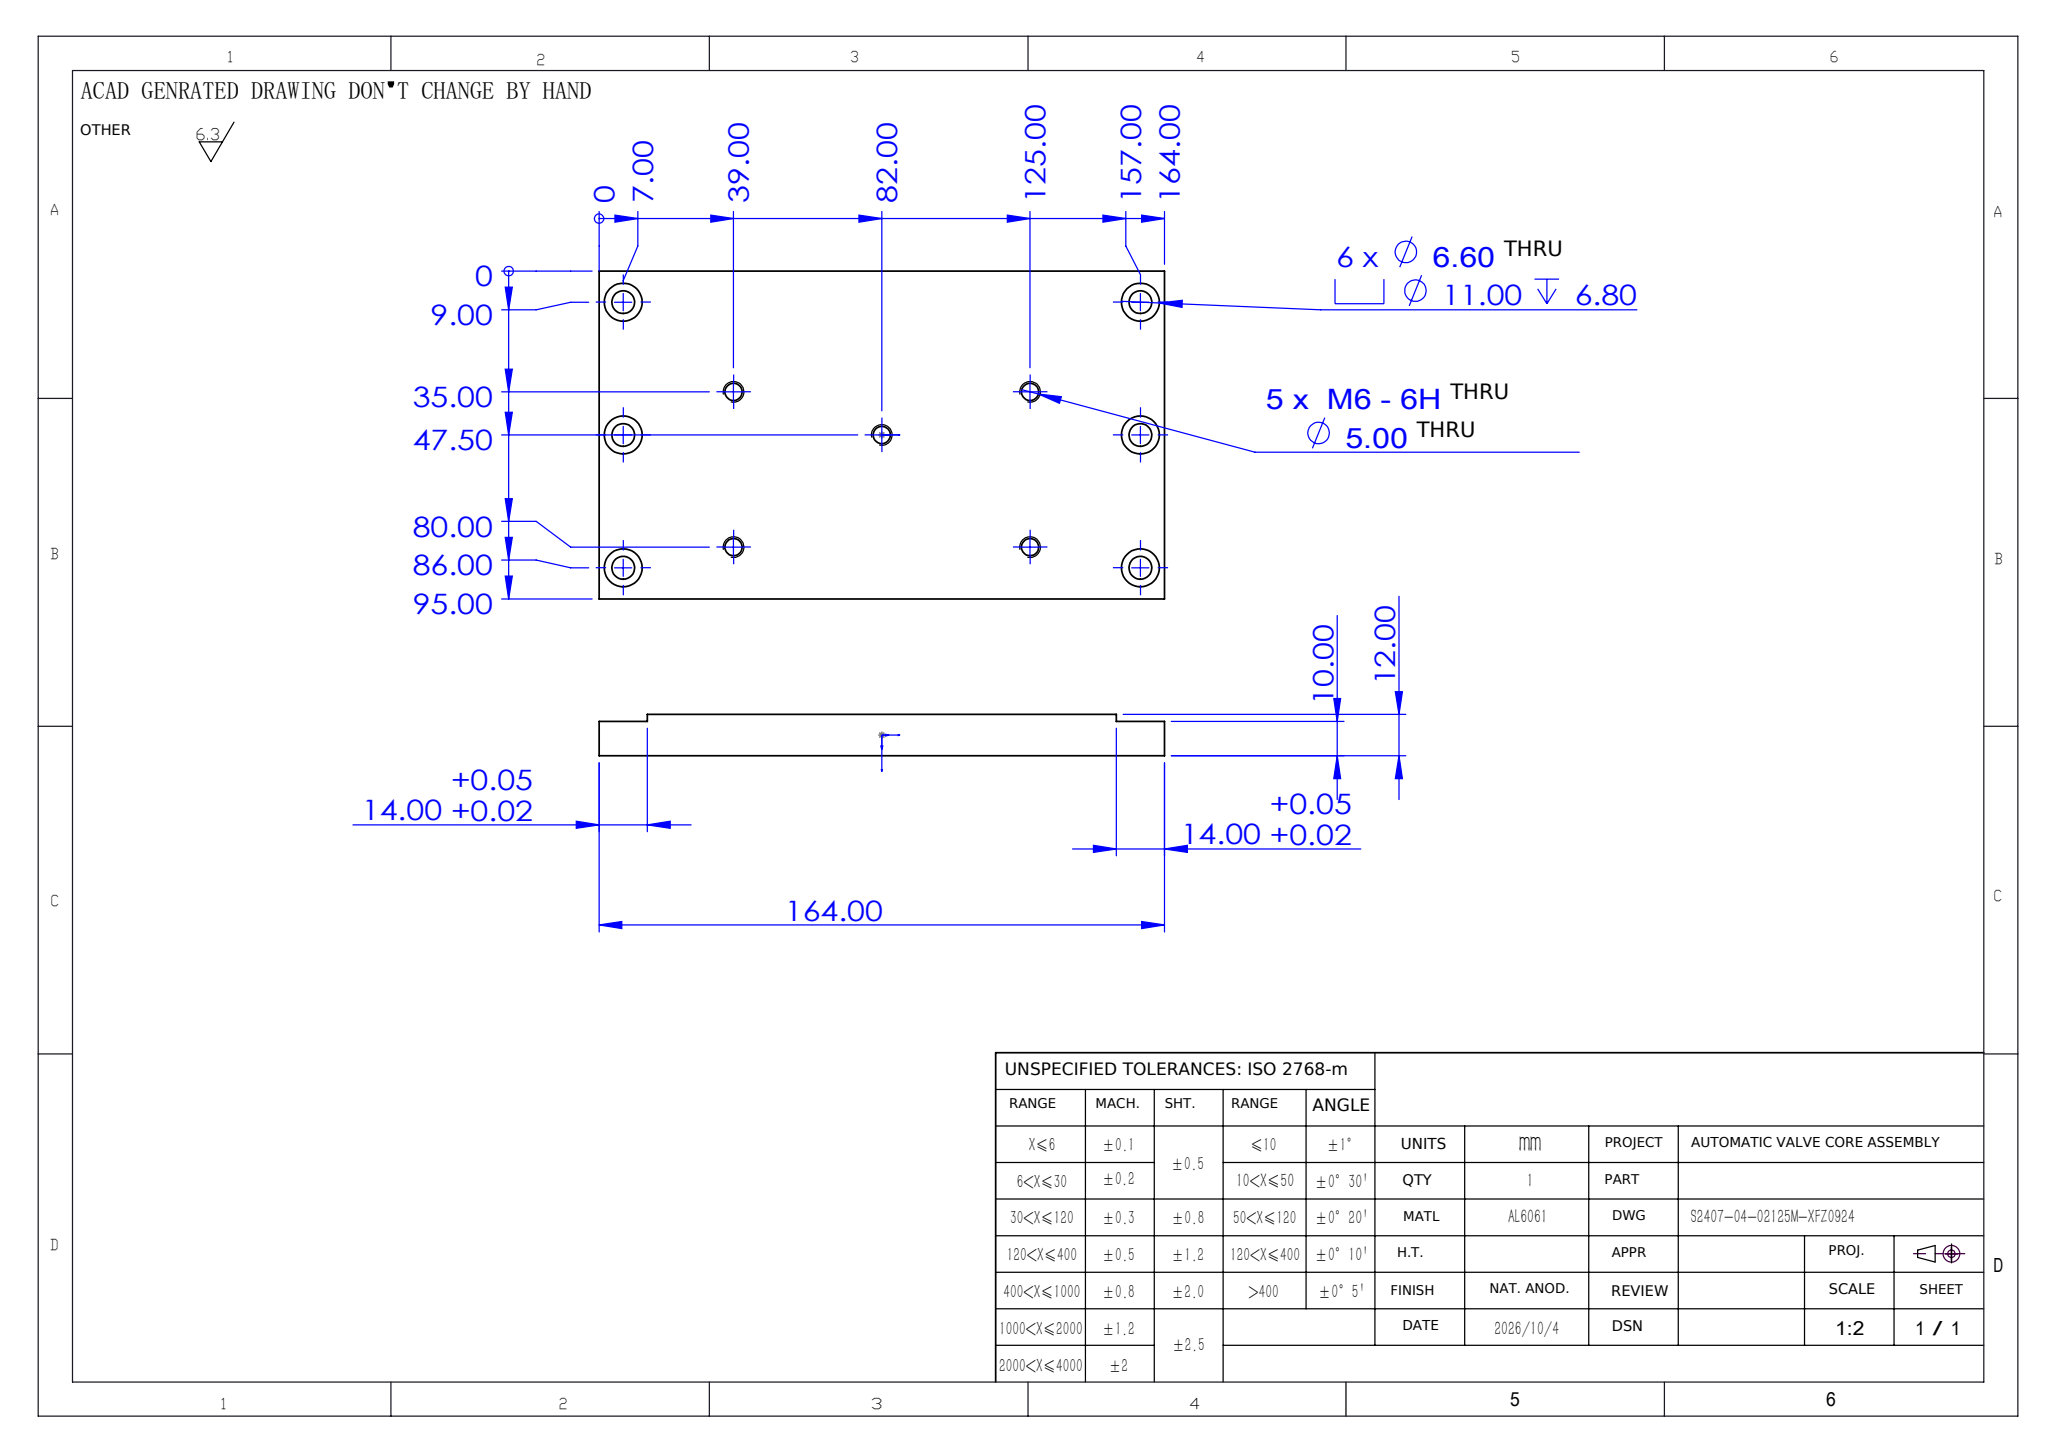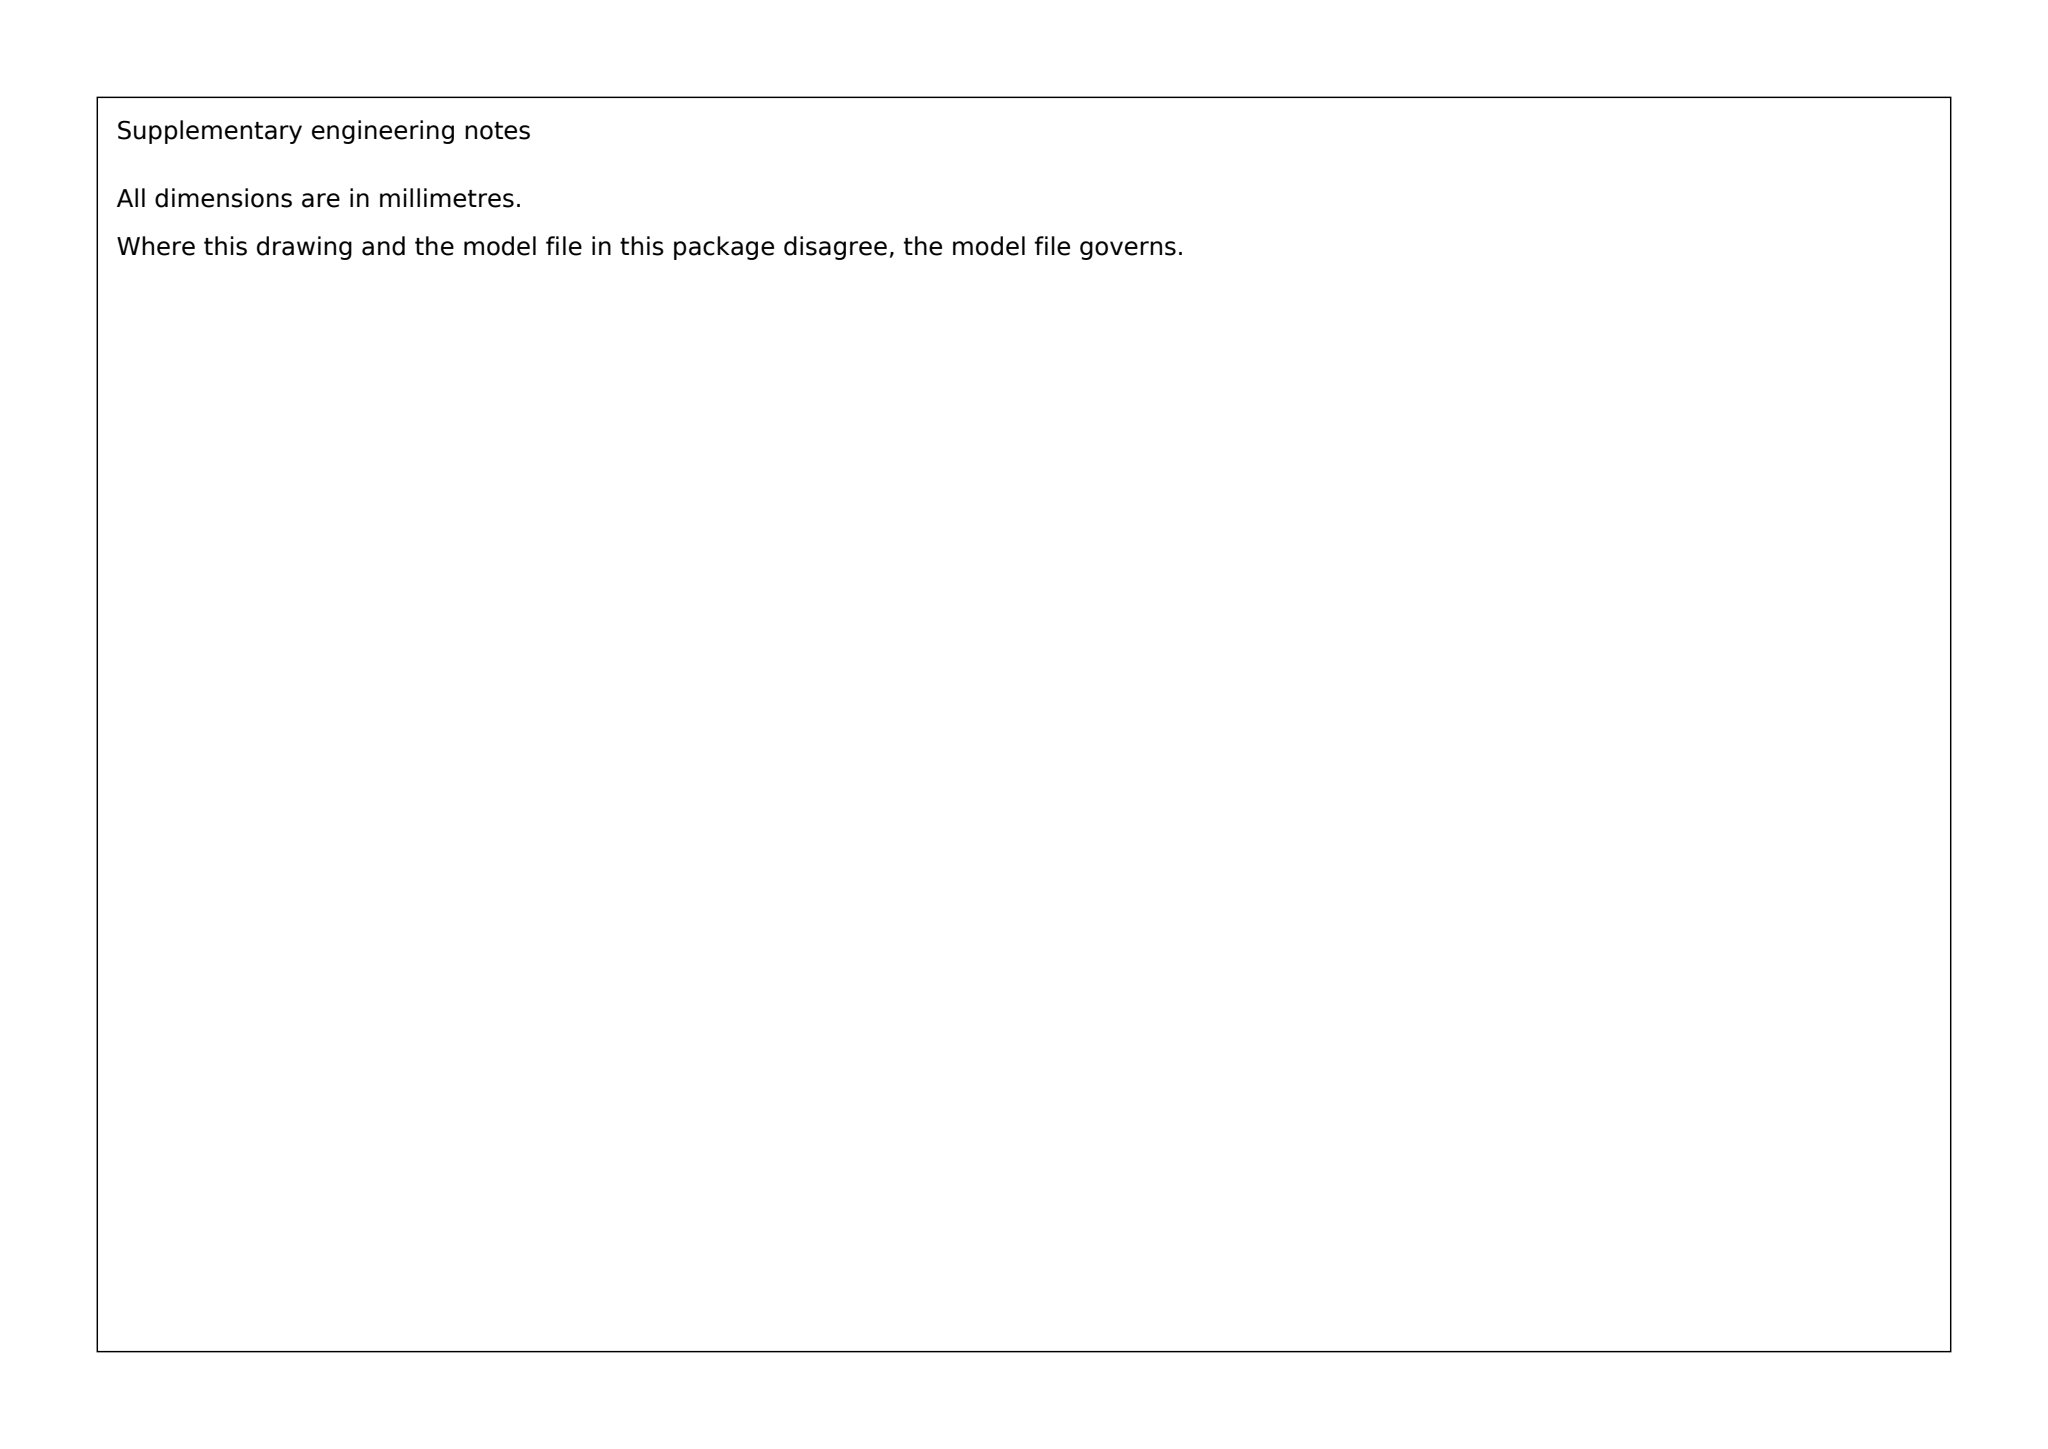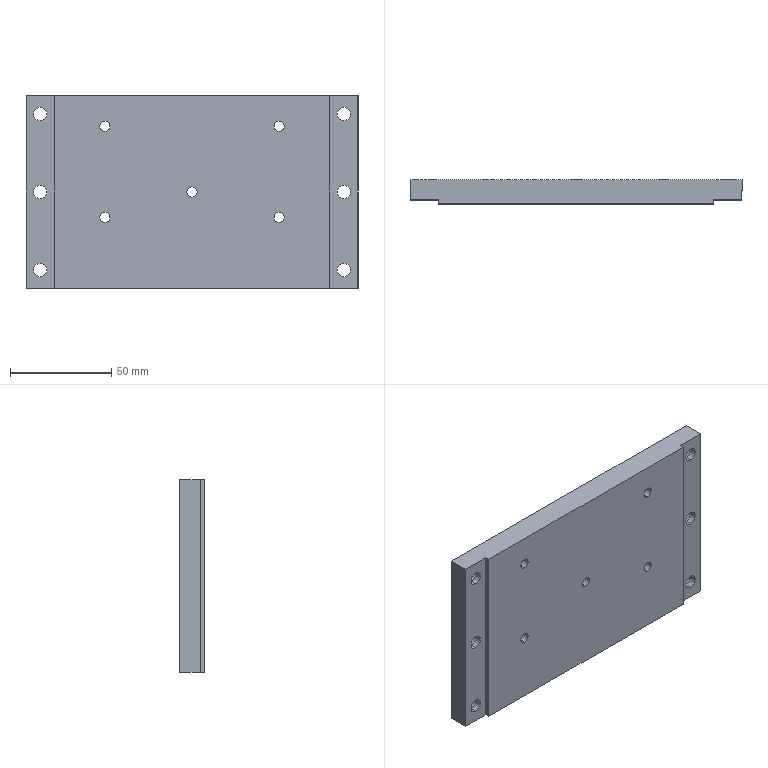Part | SolidWorks | mm | 1 solid | 50 faces | box 164 x 12 x 95 mm | volume 175928 mm3 | cylinder 34 | plane 16 | commonest cylinder face diameters 11 x12 6.6 x12 5 x10
build123d program:
from build123d import *

# Parameters (mm, degrees)
SKETCH1_W                                          = 164
SKETCH1_H                                          = 95
BOSS_EXTRUDE1_DEPTH                                = 6
M6_TAPPED_HOLE1_D                                  = 5
SKETCH4_W                                          = 14
SKETCH4_H                                          = 95
CUT_EXTRUDE1_DEPTH                                 = 2
HOLE_SIZE_ACCORDING_TO_TYPE_1_OF_HEXAG_D           = 6.6
HOLE_SIZE_ACCORDING_TO_TYPE_1_OF_HEXAG_CBORE_D     = 11
HOLE_SIZE_ACCORDING_TO_TYPE_1_OF_HEXAG_CBORE_DEPTH = 6.8


with BuildPart() as part:
    # Sketch1 → Boss-Extrude1 (new, symmetric)
    with BuildSketch(Plane(origin=(0, 0, 0), x_dir=(1, 0, 0), z_dir=(0, 1, 0))):
        Rectangle(SKETCH1_W, SKETCH1_H)
    extrude(amount=BOSS_EXTRUDE1_DEPTH, both=True)

    # M6 Tapped Hole1 (through all)
    with Locations(Plane(origin=(0, 6, 0), x_dir=(1, 0, 0), z_dir=(0, 1, 0))):
        with Locations((0, 0), (-43, -32.5), (43, -32.5), (-43, 12.5), (43, 12.5)):
            Hole(M6_TAPPED_HOLE1_D / 2)

    # Sketch4 → Cut-Extrude1 (cut)
    with BuildSketch(Plane.XZ.offset(6)):
        with Locations((-75, 0)):
            Rectangle(SKETCH4_W, SKETCH4_H)
        with Locations((75, 0)):
            Rectangle(SKETCH4_W, SKETCH4_H)
    extrude(amount=-CUT_EXTRUDE1_DEPTH, mode=Mode.SUBTRACT)

    # Hole Size _According to_ Type 1 of Hexag (through all)
    with Locations(Plane(origin=(0, 6, 0), x_dir=(1, 0, 0), z_dir=(0, 1, 0))):
        with Locations((75, 38.5), (-75, 38.5), (-75, -38.5), (-75, 0), (75, 0), (75, -38.5)):
            CounterBoreHole(HOLE_SIZE_ACCORDING_TO_TYPE_1_OF_HEXAG_D / 2, HOLE_SIZE_ACCORDING_TO_TYPE_1_OF_HEXAG_CBORE_D / 2, HOLE_SIZE_ACCORDING_TO_TYPE_1_OF_HEXAG_CBORE_DEPTH)


solid = part.part